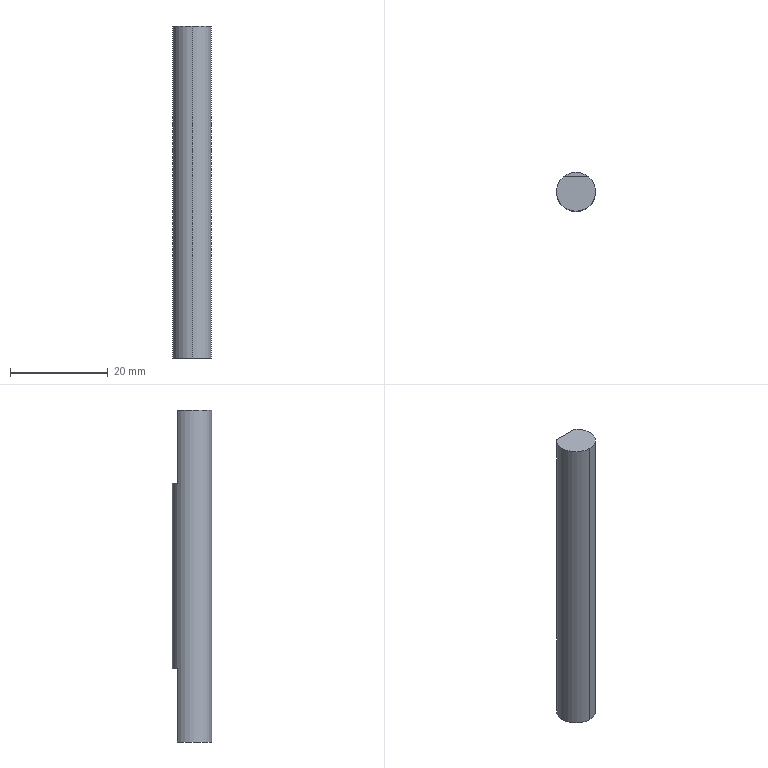Component | SolidWorks | --MA18S200418mmSolderingIron-1 | 1 solid | 8 faces | box 8 x 8 x 68 mm | volume 3309 mm3 | plane 6 | cylinder 2 | commonest cylinder face diameters 8 x2
build123d program:
from build123d import *

# Parameters (mm, degrees)
SKETCH1_R           = 4
BOSS_EXTRUDE1_DEPTH = 68
SKETCH2_W           = 4.184
SKETCH2_H           = 10.917
CUT_EXTRUDE1_DEPTH  = 15
SKETCH3_W           = 3.437
SKETCH3_H           = 7.918
CUT_EXTRUDE2_DEPTH  = 15


with BuildPart() as part:
    # Sketch1 → Boss-Extrude1 (new body)
    with BuildSketch(Plane.XY):
        Circle(SKETCH1_R)
    extrude(amount=BOSS_EXTRUDE1_DEPTH)

    # Sketch2 → Cut-Extrude1 (cut)
    with BuildSketch(Plane.XY.offset(68)):
        with Locations((-5.092, 0.1202)):
            Rectangle(SKETCH2_W, SKETCH2_H)
    extrude(amount=-CUT_EXTRUDE1_DEPTH, mode=Mode.SUBTRACT)

    # Sketch3 → Cut-Extrude2 (cut)
    with BuildSketch(Plane(origin=(0, 0, 0), x_dir=(-1, 0, 0), z_dir=(0, 0, -1))):
        with Locations((4.719, 0.0487)):
            Rectangle(SKETCH3_W, SKETCH3_H)
    extrude(amount=-CUT_EXTRUDE2_DEPTH, mode=Mode.SUBTRACT)


solid = part.part

# Placed as in the assembly
solid = solid.moved(Location((-165.956, 96.699, 0), (0, 0, -90)))
STEP:
#1=COLOUR_RGB('',0.7922,0.8196,0.9333);
#2=FILL_AREA_STYLE_COLOUR('',#1);
#3=FILL_AREA_STYLE('',(#2));
#4=SURFACE_STYLE_FILL_AREA(#3);
#5=SURFACE_SIDE_STYLE('',(#4));
#6=SURFACE_STYLE_USAGE(.BOTH.,#5);
#7=PRESENTATION_STYLE_ASSIGNMENT((#6));
#8=CARTESIAN_POINT('',(-6.534,3.65,2.677));
#9=VERTEX_POINT('',#8);
#10=CARTESIAN_POINT('',(-6.43,3.925,2.677));
#11=VERTEX_POINT('',#10);
#12=CARTESIAN_POINT('',(-6.534,3.807,2.677));
#13=DIRECTION('',(0.,0.,1.));
#14=DIRECTION('',(0.,-1.,0.));
#15=AXIS2_PLACEMENT_3D('',#12,#13,#14);
#16=CIRCLE('',#15,0.1575);
#17=EDGE_CURVE('',#9,#11,#16,.T.);
#18=ORIENTED_EDGE('',*,*,#17,.F.);
#19=CARTESIAN_POINT('',(-6.534,3.65,0.));
#20=VERTEX_POINT('',#19);
#21=CARTESIAN_POINT('',(-6.534,3.65,2.677));
#22=DIRECTION('',(0.,0.,-1.));
#23=VECTOR('',#22,39.37);
#24=LINE('',#21,#23);
#25=EDGE_CURVE('',#9,#20,#24,.T.);
#26=ORIENTED_EDGE('',*,*,#25,.T.);
#27=CARTESIAN_POINT('',(-6.43,3.925,0.));
#28=VERTEX_POINT('',#27);
#29=CARTESIAN_POINT('',(-6.534,3.807,0.));
#30=DIRECTION('',(0.,0.,1.));
#31=DIRECTION('',(0.,-1.,0.));
#32=AXIS2_PLACEMENT_3D('',#29,#30,#31);
#33=CIRCLE('',#32,0.1575);
#34=EDGE_CURVE('',#20,#28,#33,.T.);
#35=ORIENTED_EDGE('',*,*,#34,.T.);
#36=CARTESIAN_POINT('',(-6.43,3.925,0.5906));
#37=VERTEX_POINT('',#36);
#38=CARTESIAN_POINT('',(-6.43,3.925,2.677));
#39=DIRECTION('',(0.,0.,1.));
#40=VECTOR('',#39,39.37);
#41=LINE('',#38,#40);
#42=EDGE_CURVE('',#28,#37,#41,.T.);
#43=ORIENTED_EDGE('',*,*,#42,.T.);
#44=CARTESIAN_POINT('',(-6.534,3.965,0.5906));
#45=VERTEX_POINT('',#44);
#46=CARTESIAN_POINT('',(-6.534,3.807,0.5906));
#47=DIRECTION('',(0.,0.,-1.));
#48=DIRECTION('',(0.,1.,0.));
#49=AXIS2_PLACEMENT_3D('',#46,#47,#48);
#50=CIRCLE('',#49,0.1575);
#51=EDGE_CURVE('',#45,#37,#50,.T.);
#52=ORIENTED_EDGE('',*,*,#51,.F.);
#53=CARTESIAN_POINT('',(-6.534,3.965,2.087));
#54=VERTEX_POINT('',#53);
#55=CARTESIAN_POINT('',(-6.534,3.965,2.677));
#56=DIRECTION('',(0.,0.,-1.));
#57=VECTOR('',#56,39.37);
#58=LINE('',#55,#57);
#59=EDGE_CURVE('',#54,#45,#58,.T.);
#60=ORIENTED_EDGE('',*,*,#59,.F.);
#61=CARTESIAN_POINT('',(-6.43,3.925,2.087));
#62=VERTEX_POINT('',#61);
#63=CARTESIAN_POINT('',(-6.534,3.807,2.087));
#64=DIRECTION('',(0.,0.,1.));
#65=DIRECTION('',(0.,-1.,0.));
#66=AXIS2_PLACEMENT_3D('',#63,#64,#65);
#67=CIRCLE('',#66,0.1575);
#68=EDGE_CURVE('',#62,#54,#67,.T.);
#69=ORIENTED_EDGE('',*,*,#68,.F.);
#70=CARTESIAN_POINT('',(-6.43,3.925,2.677));
#71=DIRECTION('',(0.,0.,1.));
#72=VECTOR('',#71,39.37);
#73=LINE('',#70,#72);
#74=EDGE_CURVE('',#62,#11,#73,.T.);
#75=ORIENTED_EDGE('',*,*,#74,.T.);
#76=EDGE_LOOP('',(#18,#26,#35,#43,#52,#60,#69,#75));
#77=FACE_OUTER_BOUND('',#76,.T.);
#78=CARTESIAN_POINT('',(-6.534,3.807,2.677));
#79=DIRECTION('',(0.,0.,-1.));
#80=DIRECTION('',(0.,1.,0.));
#81=AXIS2_PLACEMENT_3D('',#78,#79,#80);
#82=CYLINDRICAL_SURFACE('',#81,0.1575);
#83=ADVANCED_FACE('',(#77),#82,.T.);
#84=ORIENTED_EDGE('',*,*,#25,.F.);
#85=CARTESIAN_POINT('',(-6.638,3.925,2.677));
#86=VERTEX_POINT('',#85);
#87=CARTESIAN_POINT('',(-6.534,3.807,2.677));
#88=DIRECTION('',(0.,0.,1.));
#89=DIRECTION('',(0.,-1.,0.));
#90=AXIS2_PLACEMENT_3D('',#87,#88,#89);
#91=CIRCLE('',#90,0.1575);
#92=EDGE_CURVE('',#86,#9,#91,.T.);
#93=ORIENTED_EDGE('',*,*,#92,.F.);
#94=CARTESIAN_POINT('',(-6.638,3.925,2.087));
#95=VERTEX_POINT('',#94);
#96=CARTESIAN_POINT('',(-6.638,3.925,2.677));
#97=DIRECTION('',(0.,0.,-1.));
#98=VECTOR('',#97,39.37);
#99=LINE('',#96,#98);
#100=EDGE_CURVE('',#86,#95,#99,.T.);
#101=ORIENTED_EDGE('',*,*,#100,.T.);
#102=CARTESIAN_POINT('',(-6.534,3.807,2.087));
#103=DIRECTION('',(0.,0.,1.));
#104=DIRECTION('',(0.,-1.,0.));
#105=AXIS2_PLACEMENT_3D('',#102,#103,#104);
#106=CIRCLE('',#105,0.1575);
#107=EDGE_CURVE('',#54,#95,#106,.T.);
#108=ORIENTED_EDGE('',*,*,#107,.F.);
#109=ORIENTED_EDGE('',*,*,#59,.T.);
#110=CARTESIAN_POINT('',(-6.638,3.925,0.5906));
#111=VERTEX_POINT('',#110);
#112=CARTESIAN_POINT('',(-6.534,3.807,0.5906));
#113=DIRECTION('',(0.,0.,-1.));
#114=DIRECTION('',(0.,1.,0.));
#115=AXIS2_PLACEMENT_3D('',#112,#113,#114);
#116=CIRCLE('',#115,0.1575);
#117=EDGE_CURVE('',#111,#45,#116,.T.);
#118=ORIENTED_EDGE('',*,*,#117,.F.);
#119=CARTESIAN_POINT('',(-6.638,3.925,0.));
#120=VERTEX_POINT('',#119);
#121=CARTESIAN_POINT('',(-6.638,3.925,2.677));
#122=DIRECTION('',(0.,0.,-1.));
#123=VECTOR('',#122,39.37);
#124=LINE('',#121,#123);
#125=EDGE_CURVE('',#111,#120,#124,.T.);
#126=ORIENTED_EDGE('',*,*,#125,.T.);
#127=CARTESIAN_POINT('',(-6.534,3.807,0.));
#128=DIRECTION('',(0.,0.,1.));
#129=DIRECTION('',(0.,-1.,0.));
#130=AXIS2_PLACEMENT_3D('',#127,#128,#129);
#131=CIRCLE('',#130,0.1575);
#132=EDGE_CURVE('',#120,#20,#131,.T.);
#133=ORIENTED_EDGE('',*,*,#132,.T.);
#134=EDGE_LOOP('',(#84,#93,#101,#108,#109,#118,#126,#133));
#135=FACE_OUTER_BOUND('',#134,.T.);
#136=CARTESIAN_POINT('',(-6.534,3.807,2.677));
#137=DIRECTION('',(0.,0.,-1.));
#138=DIRECTION('',(0.,1.,0.));
#139=AXIS2_PLACEMENT_3D('',#136,#137,#138);
#140=CYLINDRICAL_SURFACE('',#139,0.1575);
#141=ADVANCED_FACE('',(#135),#140,.T.);
#142=CARTESIAN_POINT('',(-6.534,3.925,2.677));
#143=DIRECTION('',(1.,0.,0.));
#144=VECTOR('',#143,39.37);
#145=LINE('',#142,#144);
#146=EDGE_CURVE('',#86,#11,#145,.T.);
#147=ORIENTED_EDGE('',*,*,#146,.F.);
#148=ORIENTED_EDGE('',*,*,#92,.T.);
#149=ORIENTED_EDGE('',*,*,#17,.T.);
#150=EDGE_LOOP('',(#147,#148,#149));
#151=FACE_OUTER_BOUND('',#150,.T.);
#152=CARTESIAN_POINT('',(-6.534,3.807,2.677));
#153=DIRECTION('',(0.,0.,1.));
#154=DIRECTION('',(-0.,-1.,0.));
#155=AXIS2_PLACEMENT_3D('',#152,#153,#154);
#156=PLANE('',#155);
#157=ADVANCED_FACE('',(#151),#156,.T.);
#158=ORIENTED_EDGE('',*,*,#132,.F.);
#159=CARTESIAN_POINT('',(-6.534,3.925,0.));
#160=DIRECTION('',(1.,-0.,0.));
#161=VECTOR('',#160,39.37);
#162=LINE('',#159,#161);
#163=EDGE_CURVE('',#120,#28,#162,.T.);
#164=ORIENTED_EDGE('',*,*,#163,.T.);
#165=ORIENTED_EDGE('',*,*,#34,.F.);
#166=EDGE_LOOP('',(#158,#164,#165));
#167=FACE_OUTER_BOUND('',#166,.T.);
#168=CARTESIAN_POINT('',(-6.534,3.807,0.));
#169=DIRECTION('',(0.,0.,1.));
#170=DIRECTION('',(-0.,-1.,0.));
#171=AXIS2_PLACEMENT_3D('',#168,#169,#170);
#172=PLANE('',#171);
#173=ADVANCED_FACE('',(#167),#172,.F.);
#174=ORIENTED_EDGE('',*,*,#68,.T.);
#175=ORIENTED_EDGE('',*,*,#107,.T.);
#176=CARTESIAN_POINT('',(-6.314,3.925,2.087));
#177=DIRECTION('',(1.,0.,0.));
#178=VECTOR('',#177,39.37);
#179=LINE('',#176,#178);
#180=EDGE_CURVE('',#95,#62,#179,.T.);
#181=ORIENTED_EDGE('',*,*,#180,.T.);
#182=EDGE_LOOP('',(#174,#175,#181));
#183=FACE_OUTER_BOUND('',#182,.T.);
#184=CARTESIAN_POINT('',(-6.744,4.09,2.087));
#185=DIRECTION('',(0.,0.,1.));
#186=DIRECTION('',(-0.,-1.,0.));
#187=AXIS2_PLACEMENT_3D('',#184,#185,#186);
#188=PLANE('',#187);
#189=ADVANCED_FACE('',(#183),#188,.T.);
#190=ORIENTED_EDGE('',*,*,#146,.T.);
#191=ORIENTED_EDGE('',*,*,#74,.F.);
#192=ORIENTED_EDGE('',*,*,#180,.F.);
#193=ORIENTED_EDGE('',*,*,#100,.F.);
#194=EDGE_LOOP('',(#190,#191,#192,#193));
#195=FACE_OUTER_BOUND('',#194,.T.);
#196=CARTESIAN_POINT('',(-6.314,3.925,2.087));
#197=DIRECTION('',(0.,-1.,0.));
#198=DIRECTION('',(1.,0.,0.));
#199=AXIS2_PLACEMENT_3D('',#196,#197,#198);
#200=PLANE('',#199);
#201=ADVANCED_FACE('',(#195),#200,.F.);
#202=ORIENTED_EDGE('',*,*,#117,.T.);
#203=ORIENTED_EDGE('',*,*,#51,.T.);
#204=CARTESIAN_POINT('',(-6.376,3.925,0.5906));
#205=DIRECTION('',(-1.,0.,0.));
#206=VECTOR('',#205,39.37);
#207=LINE('',#204,#206);
#208=EDGE_CURVE('',#37,#111,#207,.T.);
#209=ORIENTED_EDGE('',*,*,#208,.T.);
#210=EDGE_LOOP('',(#202,#203,#209));
#211=FACE_OUTER_BOUND('',#210,.T.);
#212=CARTESIAN_POINT('',(-6.688,3.925,0.5906));
#213=DIRECTION('',(0.,0.,-1.));
#214=DIRECTION('',(0.,1.,0.));
#215=AXIS2_PLACEMENT_3D('',#212,#213,#214);
#216=PLANE('',#215);
#217=ADVANCED_FACE('',(#211),#216,.T.);
#218=ORIENTED_EDGE('',*,*,#208,.F.);
#219=ORIENTED_EDGE('',*,*,#42,.F.);
#220=ORIENTED_EDGE('',*,*,#163,.F.);
#221=ORIENTED_EDGE('',*,*,#125,.F.);
#222=EDGE_LOOP('',(#218,#219,#220,#221));
#223=FACE_OUTER_BOUND('',#222,.T.);
#224=CARTESIAN_POINT('',(-6.376,3.925,0.5906));
#225=DIRECTION('',(-0.,-1.,0.));
#226=DIRECTION('',(1.,-0.,0.));
#227=AXIS2_PLACEMENT_3D('',#224,#225,#226);
#228=PLANE('',#227);
#229=ADVANCED_FACE('',(#223),#228,.F.);
#230=CLOSED_SHELL('',(#83,#141,#157,#173,#189,#201,#217,#229));
#231=MANIFOLD_SOLID_BREP('',#230);
#232=STYLED_ITEM('',(#7),#231);
#233=PRESENTATION_LAYER_ASSIGNMENT('','',(#232));
#234=(LENGTH_UNIT()NAMED_UNIT(*)SI_UNIT($,.METRE.));
#235=LENGTH_MEASURE_WITH_UNIT(LENGTH_MEASURE(0.0254),#234);
#236=DIMENSIONAL_EXPONENTS(1.,0.,0.,0.,0.,0.,0.);
#237=(CONVERSION_BASED_UNIT('',#235)LENGTH_UNIT()NAMED_UNIT(#236));
#238=UNCERTAINTY_MEASURE_WITH_UNIT(LENGTH_MEASURE(0.00001),#237,'','');
#239=(NAMED_UNIT(*)PLANE_ANGLE_UNIT()SI_UNIT($,.RADIAN.));
#240=(NAMED_UNIT(*)SI_UNIT($,.STERADIAN.)SOLID_ANGLE_UNIT());
#241=(GEOMETRIC_REPRESENTATION_CONTEXT(3)GLOBAL_UNCERTAINTY_ASSIGNED_CONTEXT((#238))GLOBAL_UNIT_ASSIGNED_CONTEXT((#237,#239,#240))REPRESENTATION_CONTEXT('',''));
#242=MECHANICAL_DESIGN_GEOMETRIC_PRESENTATION_REPRESENTATION('',(#232),#241);
#243=CARTESIAN_POINT('',(0.,0.,0.));
#244=DIRECTION('',(0.,0.,1.));
#245=DIRECTION('',(1.,0.,0.));
#246=AXIS2_PLACEMENT_3D('',#243,#244,#245);
#247=(LENGTH_UNIT()NAMED_UNIT(*)SI_UNIT($,.METRE.));
#248=LENGTH_MEASURE_WITH_UNIT(LENGTH_MEASURE(0.0254),#247);
#249=DIMENSIONAL_EXPONENTS(1.,0.,0.,0.,0.,0.,0.);
#250=(CONVERSION_BASED_UNIT('',#248)LENGTH_UNIT()NAMED_UNIT(#249));
#251=UNCERTAINTY_MEASURE_WITH_UNIT(LENGTH_MEASURE(0.00001),#250,'','');
#252=(NAMED_UNIT(*)PLANE_ANGLE_UNIT()SI_UNIT($,.RADIAN.));
#253=(NAMED_UNIT(*)SI_UNIT($,.STERADIAN.)SOLID_ANGLE_UNIT());
#254=(GEOMETRIC_REPRESENTATION_CONTEXT(3)GLOBAL_UNCERTAINTY_ASSIGNED_CONTEXT((#251))GLOBAL_UNIT_ASSIGNED_CONTEXT((#250,#252,#253))REPRESENTATION_CONTEXT('',''));
#255=ADVANCED_BREP_SHAPE_REPRESENTATION('',(#231,#246),#254);